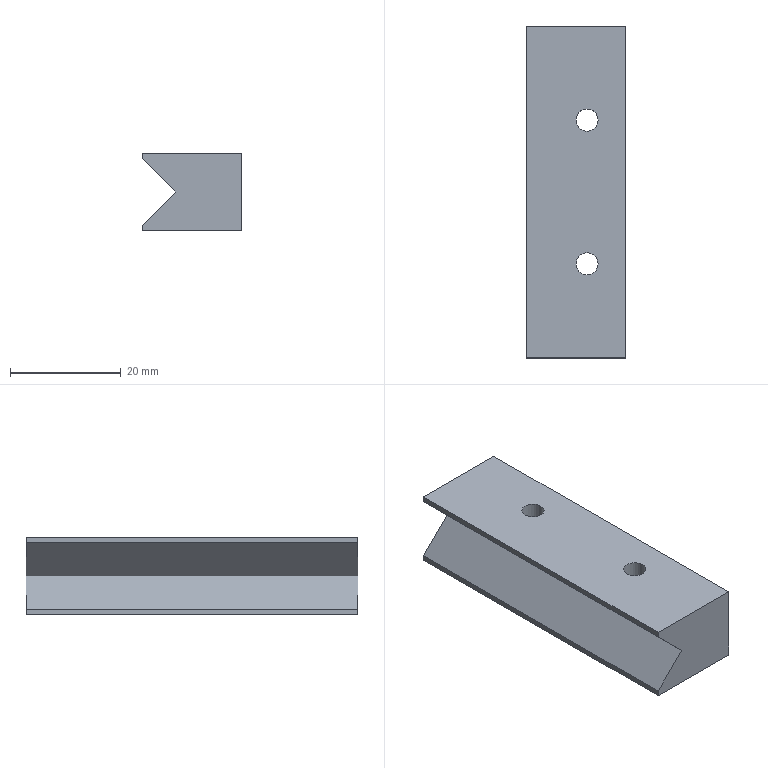Component | NX | 4_V_GUIDE | 1 solid | 15 faces | box 18 x 60 x 14 mm | volume 12264 mm3 | plane 9 | cylinder 4 | cone 2 | commonest cylinder face diameters 4 x2 4.2 x2
STEP:
#1=CARTESIAN_POINT('',(0.,0.,0.));
#2=DIRECTION('',(0.,0.,1.));
#3=DIRECTION('',(1.,0.,0.));
#4=AXIS2_PLACEMENT_3D('',#1,#2,#3);
#5=CARTESIAN_POINT('',(46.,30.,28.));
#6=VERTEX_POINT('',#5);
#7=CARTESIAN_POINT('',(46.,30.,27.));
#8=VERTEX_POINT('',#7);
#9=CARTESIAN_POINT('',(46.,30.,28.));
#10=DIRECTION('',(0.,0.,-1.));
#11=VECTOR('',#10,1.);
#12=LINE('',#9,#11);
#13=CARTESIAN_POINT('',(46.,30.,28.));
#14=DIRECTION('',(-1.,0.,0.));
#15=DIRECTION('',(0.,0.,-1.));
#16=AXIS2_PLACEMENT_3D('',#13,#14,#15);
#17=PLANE('',#16);
#18=CARTESIAN_POINT('',(0.,0.));
#19=DIRECTION('',(1.,0.));
#20=VECTOR('',#19,1.);
#21=LINE('',#18,#20);
#22=(GEOMETRIC_REPRESENTATION_CONTEXT(2)PARAMETRIC_REPRESENTATION_CONTEXT()REPRESENTATION_CONTEXT('',''));
#23=DEFINITIONAL_REPRESENTATION('',(#21),#22);
#24=PCURVE('',#17,#23);
#25=CARTESIAN_POINT('',(64.,30.,21.));
#26=DIRECTION('',(0.,-1.,0.));
#27=DIRECTION('',(-1.,0.,0.));
#28=AXIS2_PLACEMENT_3D('',#25,#26,#27);
#29=PLANE('',#28);
#30=CARTESIAN_POINT('',(18.,-7.));
#31=DIRECTION('',(0.,1.));
#32=VECTOR('',#31,1.);
#33=LINE('',#30,#32);
#34=(GEOMETRIC_REPRESENTATION_CONTEXT(2)PARAMETRIC_REPRESENTATION_CONTEXT()REPRESENTATION_CONTEXT('',''));
#35=DEFINITIONAL_REPRESENTATION('',(#33),#34);
#36=PCURVE('',#29,#35);
#37=SURFACE_CURVE('',#12,(#24,#36),.PCURVE_S1.);
#38=EDGE_CURVE('',#6,#8,#37,.T.);
#39=ORIENTED_EDGE('',*,*,#38,.T.);
#40=CARTESIAN_POINT('',(46.,-30.,27.));
#41=VERTEX_POINT('',#40);
#42=CARTESIAN_POINT('',(46.,55.,27.));
#43=DIRECTION('',(0.,-1.,0.));
#44=VECTOR('',#43,1.);
#45=LINE('',#42,#44);
#46=CARTESIAN_POINT('',(1.,-25.));
#47=DIRECTION('',(0.,1.));
#48=VECTOR('',#47,1.);
#49=LINE('',#46,#48);
#50=(GEOMETRIC_REPRESENTATION_CONTEXT(2)PARAMETRIC_REPRESENTATION_CONTEXT()REPRESENTATION_CONTEXT('',''));
#51=DEFINITIONAL_REPRESENTATION('',(#49),#50);
#52=PCURVE('',#17,#51);
#53=CARTESIAN_POINT('',(46.,55.,27.));
#54=DIRECTION('',(-0.7071,0.,-0.7071));
#55=DIRECTION('',(0.7071,0.,-0.7071));
#56=AXIS2_PLACEMENT_3D('',#53,#54,#55);
#57=PLANE('',#56);
#58=CARTESIAN_POINT('',(0.,0.));
#59=DIRECTION('',(0.,1.));
#60=VECTOR('',#59,1.);
#61=LINE('',#58,#60);
#62=(GEOMETRIC_REPRESENTATION_CONTEXT(2)PARAMETRIC_REPRESENTATION_CONTEXT()REPRESENTATION_CONTEXT('',''));
#63=DEFINITIONAL_REPRESENTATION('',(#61),#62);
#64=PCURVE('',#57,#63);
#65=SURFACE_CURVE('',#45,(#52,#64),.PCURVE_S1.);
#66=EDGE_CURVE('',#8,#41,#65,.T.);
#67=ORIENTED_EDGE('',*,*,#66,.T.);
#68=CARTESIAN_POINT('',(46.,-30.,28.));
#69=VERTEX_POINT('',#68);
#70=CARTESIAN_POINT('',(46.,-30.,28.));
#71=DIRECTION('',(0.,0.,-1.));
#72=VECTOR('',#71,1.);
#73=LINE('',#70,#72);
#74=CARTESIAN_POINT('',(0.,60.));
#75=DIRECTION('',(1.,0.));
#76=VECTOR('',#75,1.);
#77=LINE('',#74,#76);
#78=(GEOMETRIC_REPRESENTATION_CONTEXT(2)PARAMETRIC_REPRESENTATION_CONTEXT()REPRESENTATION_CONTEXT('',''));
#79=DEFINITIONAL_REPRESENTATION('',(#77),#78);
#80=PCURVE('',#17,#79);
#81=CARTESIAN_POINT('',(64.,-30.,21.));
#82=DIRECTION('',(0.,-1.,0.));
#83=DIRECTION('',(-1.,0.,0.));
#84=AXIS2_PLACEMENT_3D('',#81,#82,#83);
#85=PLANE('',#84);
#86=CARTESIAN_POINT('',(18.,-7.));
#87=DIRECTION('',(0.,1.));
#88=VECTOR('',#87,1.);
#89=LINE('',#86,#88);
#90=(GEOMETRIC_REPRESENTATION_CONTEXT(2)PARAMETRIC_REPRESENTATION_CONTEXT()REPRESENTATION_CONTEXT('',''));
#91=DEFINITIONAL_REPRESENTATION('',(#89),#90);
#92=PCURVE('',#85,#91);
#93=SURFACE_CURVE('',#73,(#80,#92),.PCURVE_S1.);
#94=EDGE_CURVE('',#69,#41,#93,.T.);
#95=ORIENTED_EDGE('',*,*,#94,.F.);
#96=CARTESIAN_POINT('',(46.,30.,28.));
#97=DIRECTION('',(0.,-1.,0.));
#98=VECTOR('',#97,1.);
#99=LINE('',#96,#98);
#100=CARTESIAN_POINT('',(0.,0.));
#101=DIRECTION('',(0.,1.));
#102=VECTOR('',#101,1.);
#103=LINE('',#100,#102);
#104=(GEOMETRIC_REPRESENTATION_CONTEXT(2)PARAMETRIC_REPRESENTATION_CONTEXT()REPRESENTATION_CONTEXT('',''));
#105=DEFINITIONAL_REPRESENTATION('',(#103),#104);
#106=PCURVE('',#17,#105);
#107=CARTESIAN_POINT('',(64.,30.,28.));
#108=DIRECTION('',(-0.,0.,1.));
#109=DIRECTION('',(-1.,0.,-0.));
#110=AXIS2_PLACEMENT_3D('',#107,#108,#109);
#111=PLANE('',#110);
#112=CARTESIAN_POINT('',(18.,0.));
#113=DIRECTION('',(0.,1.));
#114=VECTOR('',#113,1.);
#115=LINE('',#112,#114);
#116=(GEOMETRIC_REPRESENTATION_CONTEXT(2)PARAMETRIC_REPRESENTATION_CONTEXT()REPRESENTATION_CONTEXT('',''));
#117=DEFINITIONAL_REPRESENTATION('',(#115),#116);
#118=PCURVE('',#111,#117);
#119=SURFACE_CURVE('',#99,(#106,#118),.PCURVE_S1.);
#120=EDGE_CURVE('',#6,#69,#119,.T.);
#121=ORIENTED_EDGE('',*,*,#120,.F.);
#122=EDGE_LOOP('',(#39,#67,#95,#121));
#123=FACE_BOUND('',#122,.T.);
#124=ADVANCED_FACE('',(#123),#17,.T.);
#125=CARTESIAN_POINT('',(52.,30.,21.));
#126=VERTEX_POINT('',#125);
#127=CARTESIAN_POINT('',(58.,30.,15.));
#128=DIRECTION('',(0.7071,0.,-0.7071));
#129=VECTOR('',#128,1.);
#130=LINE('',#127,#129);
#131=CARTESIAN_POINT('',(6.,6.));
#132=DIRECTION('',(-0.7071,0.7071));
#133=VECTOR('',#132,1.);
#134=LINE('',#131,#133);
#135=(GEOMETRIC_REPRESENTATION_CONTEXT(2)PARAMETRIC_REPRESENTATION_CONTEXT()REPRESENTATION_CONTEXT('',''));
#136=DEFINITIONAL_REPRESENTATION('',(#134),#135);
#137=PCURVE('',#29,#136);
#138=CARTESIAN_POINT('',(16.971,25.));
#139=DIRECTION('',(1.,0.));
#140=VECTOR('',#139,1.);
#141=LINE('',#138,#140);
#142=(GEOMETRIC_REPRESENTATION_CONTEXT(2)PARAMETRIC_REPRESENTATION_CONTEXT()REPRESENTATION_CONTEXT('',''));
#143=DEFINITIONAL_REPRESENTATION('',(#141),#142);
#144=PCURVE('',#57,#143);
#145=SURFACE_CURVE('',#130,(#137,#144),.PCURVE_S1.);
#146=EDGE_CURVE('',#8,#126,#145,.T.);
#147=ORIENTED_EDGE('',*,*,#146,.F.);
#148=ORIENTED_EDGE('',*,*,#38,.F.);
#149=CARTESIAN_POINT('',(64.,30.,28.));
#150=VERTEX_POINT('',#149);
#151=CARTESIAN_POINT('',(64.,30.,28.));
#152=DIRECTION('',(-1.,0.,-0.));
#153=VECTOR('',#152,1.);
#154=LINE('',#151,#153);
#155=CARTESIAN_POINT('',(0.,-7.));
#156=DIRECTION('',(1.,0.));
#157=VECTOR('',#156,1.);
#158=LINE('',#155,#157);
#159=(GEOMETRIC_REPRESENTATION_CONTEXT(2)PARAMETRIC_REPRESENTATION_CONTEXT()REPRESENTATION_CONTEXT('',''));
#160=DEFINITIONAL_REPRESENTATION('',(#158),#159);
#161=PCURVE('',#29,#160);
#162=CARTESIAN_POINT('',(0.,0.));
#163=DIRECTION('',(1.,0.));
#164=VECTOR('',#163,1.);
#165=LINE('',#162,#164);
#166=(GEOMETRIC_REPRESENTATION_CONTEXT(2)PARAMETRIC_REPRESENTATION_CONTEXT()REPRESENTATION_CONTEXT('',''));
#167=DEFINITIONAL_REPRESENTATION('',(#165),#166);
#168=PCURVE('',#111,#167);
#169=SURFACE_CURVE('',#154,(#161,#168),.PCURVE_S1.);
#170=EDGE_CURVE('',#150,#6,#169,.T.);
#171=ORIENTED_EDGE('',*,*,#170,.F.);
#172=CARTESIAN_POINT('',(64.,30.,14.));
#173=VERTEX_POINT('',#172);
#174=CARTESIAN_POINT('',(64.,30.,14.));
#175=DIRECTION('',(0.,0.,1.));
#176=VECTOR('',#175,1.);
#177=LINE('',#174,#176);
#178=CARTESIAN_POINT('',(0.,7.));
#179=DIRECTION('',(-0.,-1.));
#180=VECTOR('',#179,1.);
#181=LINE('',#178,#180);
#182=(GEOMETRIC_REPRESENTATION_CONTEXT(2)PARAMETRIC_REPRESENTATION_CONTEXT()REPRESENTATION_CONTEXT('',''));
#183=DEFINITIONAL_REPRESENTATION('',(#181),#182);
#184=PCURVE('',#29,#183);
#185=CARTESIAN_POINT('',(64.,30.,14.));
#186=DIRECTION('',(1.,0.,-0.));
#187=DIRECTION('',(0.,0.,1.));
#188=AXIS2_PLACEMENT_3D('',#185,#186,#187);
#189=PLANE('',#188);
#190=CARTESIAN_POINT('',(0.,0.));
#191=DIRECTION('',(1.,0.));
#192=VECTOR('',#191,1.);
#193=LINE('',#190,#192);
#194=(GEOMETRIC_REPRESENTATION_CONTEXT(2)PARAMETRIC_REPRESENTATION_CONTEXT()REPRESENTATION_CONTEXT('',''));
#195=DEFINITIONAL_REPRESENTATION('',(#193),#194);
#196=PCURVE('',#189,#195);
#197=SURFACE_CURVE('',#177,(#184,#196),.PCURVE_S1.);
#198=EDGE_CURVE('',#173,#150,#197,.T.);
#199=ORIENTED_EDGE('',*,*,#198,.F.);
#200=CARTESIAN_POINT('',(46.,30.,14.));
#201=VERTEX_POINT('',#200);
#202=CARTESIAN_POINT('',(46.,30.,14.));
#203=DIRECTION('',(1.,0.,-0.));
#204=VECTOR('',#203,1.);
#205=LINE('',#202,#204);
#206=CARTESIAN_POINT('',(18.,7.));
#207=DIRECTION('',(-1.,0.));
#208=VECTOR('',#207,1.);
#209=LINE('',#206,#208);
#210=(GEOMETRIC_REPRESENTATION_CONTEXT(2)PARAMETRIC_REPRESENTATION_CONTEXT()REPRESENTATION_CONTEXT('',''));
#211=DEFINITIONAL_REPRESENTATION('',(#209),#210);
#212=PCURVE('',#29,#211);
#213=CARTESIAN_POINT('',(46.,30.,14.));
#214=DIRECTION('',(-0.,0.,-1.));
#215=DIRECTION('',(1.,0.,-0.));
#216=AXIS2_PLACEMENT_3D('',#213,#214,#215);
#217=PLANE('',#216);
#218=CARTESIAN_POINT('',(0.,0.));
#219=DIRECTION('',(1.,0.));
#220=VECTOR('',#219,1.);
#221=LINE('',#218,#220);
#222=(GEOMETRIC_REPRESENTATION_CONTEXT(2)PARAMETRIC_REPRESENTATION_CONTEXT()REPRESENTATION_CONTEXT('',''));
#223=DEFINITIONAL_REPRESENTATION('',(#221),#222);
#224=PCURVE('',#217,#223);
#225=SURFACE_CURVE('',#205,(#212,#224),.PCURVE_S1.);
#226=EDGE_CURVE('',#201,#173,#225,.T.);
#227=ORIENTED_EDGE('',*,*,#226,.F.);
#228=CARTESIAN_POINT('',(46.,30.,15.));
#229=VERTEX_POINT('',#228);
#230=CARTESIAN_POINT('',(46.,30.,28.));
#231=DIRECTION('',(0.,0.,-1.));
#232=VECTOR('',#231,1.);
#233=LINE('',#230,#232);
#234=CARTESIAN_POINT('',(18.,-7.));
#235=DIRECTION('',(0.,1.));
#236=VECTOR('',#235,1.);
#237=LINE('',#234,#236);
#238=(GEOMETRIC_REPRESENTATION_CONTEXT(2)PARAMETRIC_REPRESENTATION_CONTEXT()REPRESENTATION_CONTEXT('',''));
#239=DEFINITIONAL_REPRESENTATION('',(#237),#238);
#240=PCURVE('',#29,#239);
#241=CARTESIAN_POINT('',(46.,30.,28.));
#242=DIRECTION('',(-1.,0.,0.));
#243=DIRECTION('',(0.,0.,-1.));
#244=AXIS2_PLACEMENT_3D('',#241,#242,#243);
#245=PLANE('',#244);
#246=CARTESIAN_POINT('',(0.,0.));
#247=DIRECTION('',(1.,0.));
#248=VECTOR('',#247,1.);
#249=LINE('',#246,#248);
#250=(GEOMETRIC_REPRESENTATION_CONTEXT(2)PARAMETRIC_REPRESENTATION_CONTEXT()REPRESENTATION_CONTEXT('',''));
#251=DEFINITIONAL_REPRESENTATION('',(#249),#250);
#252=PCURVE('',#245,#251);
#253=SURFACE_CURVE('',#233,(#240,#252),.PCURVE_S1.);
#254=EDGE_CURVE('',#229,#201,#253,.T.);
#255=ORIENTED_EDGE('',*,*,#254,.F.);
#256=CARTESIAN_POINT('',(58.,30.,27.));
#257=DIRECTION('',(-0.7071,0.,-0.7071));
#258=VECTOR('',#257,1.);
#259=LINE('',#256,#258);
#260=CARTESIAN_POINT('',(6.,-6.));
#261=DIRECTION('',(0.7071,0.7071));
#262=VECTOR('',#261,1.);
#263=LINE('',#260,#262);
#264=(GEOMETRIC_REPRESENTATION_CONTEXT(2)PARAMETRIC_REPRESENTATION_CONTEXT()REPRESENTATION_CONTEXT('',''));
#265=DEFINITIONAL_REPRESENTATION('',(#263),#264);
#266=PCURVE('',#29,#265);
#267=CARTESIAN_POINT('',(52.,55.,21.));
#268=DIRECTION('',(-0.7071,0.,0.7071));
#269=DIRECTION('',(-0.7071,0.,-0.7071));
#270=AXIS2_PLACEMENT_3D('',#267,#268,#269);
#271=PLANE('',#270);
#272=CARTESIAN_POINT('',(-8.485,25.));
#273=DIRECTION('',(1.,0.));
#274=VECTOR('',#273,1.);
#275=LINE('',#272,#274);
#276=(GEOMETRIC_REPRESENTATION_CONTEXT(2)PARAMETRIC_REPRESENTATION_CONTEXT()REPRESENTATION_CONTEXT('',''));
#277=DEFINITIONAL_REPRESENTATION('',(#275),#276);
#278=PCURVE('',#271,#277);
#279=SURFACE_CURVE('',#259,(#266,#278),.PCURVE_S1.);
#280=EDGE_CURVE('',#126,#229,#279,.T.);
#281=ORIENTED_EDGE('',*,*,#280,.F.);
#282=EDGE_LOOP('',(#147,#148,#171,#199,#227,#255,#281));
#283=FACE_BOUND('',#282,.T.);
#284=ADVANCED_FACE('',(#283),#29,.F.);
#285=ORIENTED_EDGE('',*,*,#94,.T.);
#286=CARTESIAN_POINT('',(52.,-30.,21.));
#287=VERTEX_POINT('',#286);
#288=CARTESIAN_POINT('',(58.,-30.,15.));
#289=DIRECTION('',(0.7071,0.,-0.7071));
#290=VECTOR('',#289,1.);
#291=LINE('',#288,#290);
#292=CARTESIAN_POINT('',(6.,6.));
#293=DIRECTION('',(-0.7071,0.7071));
#294=VECTOR('',#293,1.);
#295=LINE('',#292,#294);
#296=(GEOMETRIC_REPRESENTATION_CONTEXT(2)PARAMETRIC_REPRESENTATION_CONTEXT()REPRESENTATION_CONTEXT('',''));
#297=DEFINITIONAL_REPRESENTATION('',(#295),#296);
#298=PCURVE('',#85,#297);
#299=CARTESIAN_POINT('',(16.971,85.));
#300=DIRECTION('',(1.,0.));
#301=VECTOR('',#300,1.);
#302=LINE('',#299,#301);
#303=(GEOMETRIC_REPRESENTATION_CONTEXT(2)PARAMETRIC_REPRESENTATION_CONTEXT()REPRESENTATION_CONTEXT('',''));
#304=DEFINITIONAL_REPRESENTATION('',(#302),#303);
#305=PCURVE('',#57,#304);
#306=SURFACE_CURVE('',#291,(#298,#305),.PCURVE_S1.);
#307=EDGE_CURVE('',#41,#287,#306,.T.);
#308=ORIENTED_EDGE('',*,*,#307,.T.);
#309=CARTESIAN_POINT('',(46.,-30.,15.));
#310=VERTEX_POINT('',#309);
#311=CARTESIAN_POINT('',(58.,-30.,27.));
#312=DIRECTION('',(-0.7071,0.,-0.7071));
#313=VECTOR('',#312,1.);
#314=LINE('',#311,#313);
#315=CARTESIAN_POINT('',(6.,-6.));
#316=DIRECTION('',(0.7071,0.7071));
#317=VECTOR('',#316,1.);
#318=LINE('',#315,#317);
#319=(GEOMETRIC_REPRESENTATION_CONTEXT(2)PARAMETRIC_REPRESENTATION_CONTEXT()REPRESENTATION_CONTEXT('',''));
#320=DEFINITIONAL_REPRESENTATION('',(#318),#319);
#321=PCURVE('',#85,#320);
#322=CARTESIAN_POINT('',(-8.485,85.));
#323=DIRECTION('',(1.,0.));
#324=VECTOR('',#323,1.);
#325=LINE('',#322,#324);
#326=(GEOMETRIC_REPRESENTATION_CONTEXT(2)PARAMETRIC_REPRESENTATION_CONTEXT()REPRESENTATION_CONTEXT('',''));
#327=DEFINITIONAL_REPRESENTATION('',(#325),#326);
#328=PCURVE('',#271,#327);
#329=SURFACE_CURVE('',#314,(#321,#328),.PCURVE_S1.);
#330=EDGE_CURVE('',#287,#310,#329,.T.);
#331=ORIENTED_EDGE('',*,*,#330,.T.);
#332=CARTESIAN_POINT('',(46.,-30.,14.));
#333=VERTEX_POINT('',#332);
#334=CARTESIAN_POINT('',(46.,-30.,28.));
#335=DIRECTION('',(0.,0.,-1.));
#336=VECTOR('',#335,1.);
#337=LINE('',#334,#336);
#338=CARTESIAN_POINT('',(18.,-7.));
#339=DIRECTION('',(0.,1.));
#340=VECTOR('',#339,1.);
#341=LINE('',#338,#340);
#342=(GEOMETRIC_REPRESENTATION_CONTEXT(2)PARAMETRIC_REPRESENTATION_CONTEXT()REPRESENTATION_CONTEXT('',''));
#343=DEFINITIONAL_REPRESENTATION('',(#341),#342);
#344=PCURVE('',#85,#343);
#345=CARTESIAN_POINT('',(0.,60.));
#346=DIRECTION('',(1.,0.));
#347=VECTOR('',#346,1.);
#348=LINE('',#345,#347);
#349=(GEOMETRIC_REPRESENTATION_CONTEXT(2)PARAMETRIC_REPRESENTATION_CONTEXT()REPRESENTATION_CONTEXT('',''));
#350=DEFINITIONAL_REPRESENTATION('',(#348),#349);
#351=PCURVE('',#245,#350);
#352=SURFACE_CURVE('',#337,(#344,#351),.PCURVE_S1.);
#353=EDGE_CURVE('',#310,#333,#352,.T.);
#354=ORIENTED_EDGE('',*,*,#353,.T.);
#355=CARTESIAN_POINT('',(64.,-30.,14.));
#356=VERTEX_POINT('',#355);
#357=CARTESIAN_POINT('',(46.,-30.,14.));
#358=DIRECTION('',(1.,0.,-0.));
#359=VECTOR('',#358,1.);
#360=LINE('',#357,#359);
#361=CARTESIAN_POINT('',(18.,7.));
#362=DIRECTION('',(-1.,0.));
#363=VECTOR('',#362,1.);
#364=LINE('',#361,#363);
#365=(GEOMETRIC_REPRESENTATION_CONTEXT(2)PARAMETRIC_REPRESENTATION_CONTEXT()REPRESENTATION_CONTEXT('',''));
#366=DEFINITIONAL_REPRESENTATION('',(#364),#365);
#367=PCURVE('',#85,#366);
#368=CARTESIAN_POINT('',(0.,60.));
#369=DIRECTION('',(1.,0.));
#370=VECTOR('',#369,1.);
#371=LINE('',#368,#370);
#372=(GEOMETRIC_REPRESENTATION_CONTEXT(2)PARAMETRIC_REPRESENTATION_CONTEXT()REPRESENTATION_CONTEXT('',''));
#373=DEFINITIONAL_REPRESENTATION('',(#371),#372);
#374=PCURVE('',#217,#373);
#375=SURFACE_CURVE('',#360,(#367,#374),.PCURVE_S1.);
#376=EDGE_CURVE('',#333,#356,#375,.T.);
#377=ORIENTED_EDGE('',*,*,#376,.T.);
#378=CARTESIAN_POINT('',(64.,-30.,28.));
#379=VERTEX_POINT('',#378);
#380=CARTESIAN_POINT('',(64.,-30.,14.));
#381=DIRECTION('',(0.,0.,1.));
#382=VECTOR('',#381,1.);
#383=LINE('',#380,#382);
#384=CARTESIAN_POINT('',(0.,7.));
#385=DIRECTION('',(-0.,-1.));
#386=VECTOR('',#385,1.);
#387=LINE('',#384,#386);
#388=(GEOMETRIC_REPRESENTATION_CONTEXT(2)PARAMETRIC_REPRESENTATION_CONTEXT()REPRESENTATION_CONTEXT('',''));
#389=DEFINITIONAL_REPRESENTATION('',(#387),#388);
#390=PCURVE('',#85,#389);
#391=CARTESIAN_POINT('',(0.,60.));
#392=DIRECTION('',(1.,0.));
#393=VECTOR('',#392,1.);
#394=LINE('',#391,#393);
#395=(GEOMETRIC_REPRESENTATION_CONTEXT(2)PARAMETRIC_REPRESENTATION_CONTEXT()REPRESENTATION_CONTEXT('',''));
#396=DEFINITIONAL_REPRESENTATION('',(#394),#395);
#397=PCURVE('',#189,#396);
#398=SURFACE_CURVE('',#383,(#390,#397),.PCURVE_S1.);
#399=EDGE_CURVE('',#356,#379,#398,.T.);
#400=ORIENTED_EDGE('',*,*,#399,.T.);
#401=CARTESIAN_POINT('',(64.,-30.,28.));
#402=DIRECTION('',(-1.,0.,-0.));
#403=VECTOR('',#402,1.);
#404=LINE('',#401,#403);
#405=CARTESIAN_POINT('',(0.,-7.));
#406=DIRECTION('',(1.,0.));
#407=VECTOR('',#406,1.);
#408=LINE('',#405,#407);
#409=(GEOMETRIC_REPRESENTATION_CONTEXT(2)PARAMETRIC_REPRESENTATION_CONTEXT()REPRESENTATION_CONTEXT('',''));
#410=DEFINITIONAL_REPRESENTATION('',(#408),#409);
#411=PCURVE('',#85,#410);
#412=CARTESIAN_POINT('',(0.,60.));
#413=DIRECTION('',(1.,0.));
#414=VECTOR('',#413,1.);
#415=LINE('',#412,#414);
#416=(GEOMETRIC_REPRESENTATION_CONTEXT(2)PARAMETRIC_REPRESENTATION_CONTEXT()REPRESENTATION_CONTEXT('',''));
#417=DEFINITIONAL_REPRESENTATION('',(#415),#416);
#418=PCURVE('',#111,#417);
#419=SURFACE_CURVE('',#404,(#411,#418),.PCURVE_S1.);
#420=EDGE_CURVE('',#379,#69,#419,.T.);
#421=ORIENTED_EDGE('',*,*,#420,.T.);
#422=EDGE_LOOP('',(#285,#308,#331,#354,#377,#400,#421));
#423=FACE_BOUND('',#422,.T.);
#424=ADVANCED_FACE('',(#423),#85,.T.);
#425=CARTESIAN_POINT('',(55.,-13.,28.));
#426=VERTEX_POINT('',#425);
#427=CARTESIAN_POINT('',(57.,-13.,28.));
#428=DIRECTION('',(-0.,0.,1.));
#429=DIRECTION('',(-1.,0.,-0.));
#430=AXIS2_PLACEMENT_3D('',#427,#428,#429);
#431=CIRCLE('',#430,2.);
#432=CARTESIAN_POINT('',(7.,43.));
#433=DIRECTION('',(1.,0.));
#434=AXIS2_PLACEMENT_2D('',#432,#433);
#435=CIRCLE('',#434,2.);
#436=(GEOMETRIC_REPRESENTATION_CONTEXT(2)PARAMETRIC_REPRESENTATION_CONTEXT()REPRESENTATION_CONTEXT('',''));
#437=DEFINITIONAL_REPRESENTATION('',(#435),#436);
#438=PCURVE('',#111,#437);
#439=CARTESIAN_POINT('',(57.,-13.,14.));
#440=DIRECTION('',(0.,0.,1.));
#441=DIRECTION('',(-1.,0.,0.));
#442=AXIS2_PLACEMENT_3D('',#439,#440,#441);
#443=CYLINDRICAL_SURFACE('',#442,2.);
#444=CARTESIAN_POINT('',(0.,14.));
#445=DIRECTION('',(1.,0.));
#446=VECTOR('',#445,1.);
#447=LINE('',#444,#446);
#448=(GEOMETRIC_REPRESENTATION_CONTEXT(2)PARAMETRIC_REPRESENTATION_CONTEXT()REPRESENTATION_CONTEXT('',''));
#449=DEFINITIONAL_REPRESENTATION('',(#447),#448);
#450=PCURVE('',#443,#449);
#451=SURFACE_CURVE('',#431,(#438,#450),.PCURVE_S1.);
#452=EDGE_CURVE('',#426,#426,#451,.T.);
#453=ORIENTED_EDGE('',*,*,#452,.F.);
#454=EDGE_LOOP('',(#453));
#455=FACE_BOUND('',#454,.T.);
#456=CARTESIAN_POINT('',(55.,13.,28.));
#457=VERTEX_POINT('',#456);
#458=CARTESIAN_POINT('',(57.,13.,28.));
#459=DIRECTION('',(-0.,0.,1.));
#460=DIRECTION('',(-1.,0.,-0.));
#461=AXIS2_PLACEMENT_3D('',#458,#459,#460);
#462=CIRCLE('',#461,2.);
#463=CARTESIAN_POINT('',(7.,17.));
#464=DIRECTION('',(1.,0.));
#465=AXIS2_PLACEMENT_2D('',#463,#464);
#466=CIRCLE('',#465,2.);
#467=(GEOMETRIC_REPRESENTATION_CONTEXT(2)PARAMETRIC_REPRESENTATION_CONTEXT()REPRESENTATION_CONTEXT('',''));
#468=DEFINITIONAL_REPRESENTATION('',(#466),#467);
#469=PCURVE('',#111,#468);
#470=CARTESIAN_POINT('',(57.,13.,14.));
#471=DIRECTION('',(0.,0.,1.));
#472=DIRECTION('',(-1.,0.,0.));
#473=AXIS2_PLACEMENT_3D('',#470,#471,#472);
#474=CYLINDRICAL_SURFACE('',#473,2.);
#475=CARTESIAN_POINT('',(0.,14.));
#476=DIRECTION('',(1.,0.));
#477=VECTOR('',#476,1.);
#478=LINE('',#475,#477);
#479=(GEOMETRIC_REPRESENTATION_CONTEXT(2)PARAMETRIC_REPRESENTATION_CONTEXT()REPRESENTATION_CONTEXT('',''));
#480=DEFINITIONAL_REPRESENTATION('',(#478),#479);
#481=PCURVE('',#474,#480);
#482=SURFACE_CURVE('',#462,(#469,#481),.PCURVE_S1.);
#483=EDGE_CURVE('',#457,#457,#482,.T.);
#484=ORIENTED_EDGE('',*,*,#483,.F.);
#485=EDGE_LOOP('',(#484));
#486=FACE_BOUND('',#485,.T.);
#487=ORIENTED_EDGE('',*,*,#420,.F.);
#488=CARTESIAN_POINT('',(64.,30.,28.));
#489=DIRECTION('',(0.,-1.,0.));
#490=VECTOR('',#489,1.);
#491=LINE('',#488,#490);
#492=CARTESIAN_POINT('',(0.,0.));
#493=DIRECTION('',(0.,1.));
#494=VECTOR('',#493,1.);
#495=LINE('',#492,#494);
#496=(GEOMETRIC_REPRESENTATION_CONTEXT(2)PARAMETRIC_REPRESENTATION_CONTEXT()REPRESENTATION_CONTEXT('',''));
#497=DEFINITIONAL_REPRESENTATION('',(#495),#496);
#498=PCURVE('',#111,#497);
#499=CARTESIAN_POINT('',(14.,0.));
#500=DIRECTION('',(0.,1.));
#501=VECTOR('',#500,1.);
#502=LINE('',#499,#501);
#503=(GEOMETRIC_REPRESENTATION_CONTEXT(2)PARAMETRIC_REPRESENTATION_CONTEXT()REPRESENTATION_CONTEXT('',''));
#504=DEFINITIONAL_REPRESENTATION('',(#502),#503);
#505=PCURVE('',#189,#504);
#506=SURFACE_CURVE('',#491,(#498,#505),.PCURVE_S1.);
#507=EDGE_CURVE('',#150,#379,#506,.T.);
#508=ORIENTED_EDGE('',*,*,#507,.F.);
#509=ORIENTED_EDGE('',*,*,#170,.T.);
#510=ORIENTED_EDGE('',*,*,#120,.T.);
#511=EDGE_LOOP('',(#487,#508,#509,#510));
#512=FACE_BOUND('',#511,.T.);
#513=ADVANCED_FACE('',(#455,#486,#512),#111,.T.);
#514=CARTESIAN_POINT('',(46.,55.,15.));
#515=DIRECTION('',(0.,-1.,0.));
#516=VECTOR('',#515,1.);
#517=LINE('',#514,#516);
#518=CARTESIAN_POINT('',(13.,-25.));
#519=DIRECTION('',(0.,1.));
#520=VECTOR('',#519,1.);
#521=LINE('',#518,#520);
#522=(GEOMETRIC_REPRESENTATION_CONTEXT(2)PARAMETRIC_REPRESENTATION_CONTEXT()REPRESENTATION_CONTEXT('',''));
#523=DEFINITIONAL_REPRESENTATION('',(#521),#522);
#524=PCURVE('',#245,#523);
#525=CARTESIAN_POINT('',(8.485,0.));
#526=DIRECTION('',(0.,1.));
#527=VECTOR('',#526,1.);
#528=LINE('',#525,#527);
#529=(GEOMETRIC_REPRESENTATION_CONTEXT(2)PARAMETRIC_REPRESENTATION_CONTEXT()REPRESENTATION_CONTEXT('',''));
#530=DEFINITIONAL_REPRESENTATION('',(#528),#529);
#531=PCURVE('',#271,#530);
#532=SURFACE_CURVE('',#517,(#524,#531),.PCURVE_S1.);
#533=EDGE_CURVE('',#229,#310,#532,.T.);
#534=ORIENTED_EDGE('',*,*,#533,.F.);
#535=ORIENTED_EDGE('',*,*,#254,.T.);
#536=CARTESIAN_POINT('',(46.,30.,14.));
#537=DIRECTION('',(0.,-1.,0.));
#538=VECTOR('',#537,1.);
#539=LINE('',#536,#538);
#540=CARTESIAN_POINT('',(14.,0.));
#541=DIRECTION('',(0.,1.));
#542=VECTOR('',#541,1.);
#543=LINE('',#540,#542);
#544=(GEOMETRIC_REPRESENTATION_CONTEXT(2)PARAMETRIC_REPRESENTATION_CONTEXT()REPRESENTATION_CONTEXT('',''));
#545=DEFINITIONAL_REPRESENTATION('',(#543),#544);
#546=PCURVE('',#245,#545);
#547=CARTESIAN_POINT('',(0.,0.));
#548=DIRECTION('',(0.,1.));
#549=VECTOR('',#548,1.);
#550=LINE('',#547,#549);
#551=(GEOMETRIC_REPRESENTATION_CONTEXT(2)PARAMETRIC_REPRESENTATION_CONTEXT()REPRESENTATION_CONTEXT('',''));
#552=DEFINITIONAL_REPRESENTATION('',(#550),#551);
#553=PCURVE('',#217,#552);
#554=SURFACE_CURVE('',#539,(#546,#553),.PCURVE_S1.);
#555=EDGE_CURVE('',#201,#333,#554,.T.);
#556=ORIENTED_EDGE('',*,*,#555,.T.);
#557=ORIENTED_EDGE('',*,*,#353,.F.);
#558=EDGE_LOOP('',(#534,#535,#556,#557));
#559=FACE_BOUND('',#558,.T.);
#560=ADVANCED_FACE('',(#559),#245,.T.);
#561=CARTESIAN_POINT('',(54.9,-22.,14.));
#562=VERTEX_POINT('',#561);
#563=CARTESIAN_POINT('',(57.,-22.,14.));
#564=DIRECTION('',(0.,0.,1.));
#565=DIRECTION('',(-1.,0.,0.));
#566=AXIS2_PLACEMENT_3D('',#563,#564,#565);
#567=CIRCLE('',#566,2.1);
#568=CARTESIAN_POINT('',(8.9,52.));
#569=CARTESIAN_POINT('',(8.9,55.637));
#570=CARTESIAN_POINT('',(12.05,53.819));
#571=CARTESIAN_POINT('',(15.2,52.));
#572=CARTESIAN_POINT('',(12.05,50.181));
#573=CARTESIAN_POINT('',(8.9,48.363));
#574=CARTESIAN_POINT('',(8.9,52.));
#575=(BOUNDED_CURVE()B_SPLINE_CURVE(2,(#568,#569,#570,#571,#572,#573,#574),.UNSPECIFIED.,.T.,.F.)B_SPLINE_CURVE_WITH_KNOTS((1,2,2,2,2,1),(-2.094,0.,2.094,4.189,6.283,8.378),.UNSPECIFIED.)CURVE()GEOMETRIC_REPRESENTATION_ITEM()RATIONAL_B_SPLINE_CURVE((1.,0.5,1.,0.5,1.,0.5,1.))REPRESENTATION_ITEM(''));
#576=(GEOMETRIC_REPRESENTATION_CONTEXT(2)PARAMETRIC_REPRESENTATION_CONTEXT()REPRESENTATION_CONTEXT('',''));
#577=DEFINITIONAL_REPRESENTATION('',(#575),#576);
#578=PCURVE('',#217,#577);
#579=CARTESIAN_POINT('',(57.,-22.,14.));
#580=DIRECTION('',(0.,0.,1.));
#581=DIRECTION('',(-1.,0.,0.));
#582=AXIS2_PLACEMENT_3D('',#579,#580,#581);
#583=CYLINDRICAL_SURFACE('',#582,2.1);
#584=CARTESIAN_POINT('',(0.,-0.));
#585=DIRECTION('',(1.,0.));
#586=VECTOR('',#585,1.);
#587=LINE('',#584,#586);
#588=(GEOMETRIC_REPRESENTATION_CONTEXT(2)PARAMETRIC_REPRESENTATION_CONTEXT()REPRESENTATION_CONTEXT('',''));
#589=DEFINITIONAL_REPRESENTATION('',(#587),#588);
#590=PCURVE('',#583,#589);
#591=SURFACE_CURVE('',#567,(#578,#590),.PCURVE_S1.);
#592=EDGE_CURVE('',#562,#562,#591,.T.);
#593=ORIENTED_EDGE('',*,*,#592,.T.);
#594=EDGE_LOOP('',(#593));
#595=FACE_BOUND('',#594,.T.);
#596=CARTESIAN_POINT('',(54.9,22.,14.));
#597=VERTEX_POINT('',#596);
#598=CARTESIAN_POINT('',(57.,22.,14.));
#599=DIRECTION('',(0.,0.,1.));
#600=DIRECTION('',(-1.,0.,0.));
#601=AXIS2_PLACEMENT_3D('',#598,#599,#600);
#602=CIRCLE('',#601,2.1);
#603=CARTESIAN_POINT('',(8.9,8.));
#604=CARTESIAN_POINT('',(8.9,11.637));
#605=CARTESIAN_POINT('',(12.05,9.819));
#606=CARTESIAN_POINT('',(15.2,8.));
#607=CARTESIAN_POINT('',(12.05,6.181));
#608=CARTESIAN_POINT('',(8.9,4.363));
#609=CARTESIAN_POINT('',(8.9,8.));
#610=(BOUNDED_CURVE()B_SPLINE_CURVE(2,(#603,#604,#605,#606,#607,#608,#609),.UNSPECIFIED.,.T.,.F.)B_SPLINE_CURVE_WITH_KNOTS((1,2,2,2,2,1),(-2.094,0.,2.094,4.189,6.283,8.378),.UNSPECIFIED.)CURVE()GEOMETRIC_REPRESENTATION_ITEM()RATIONAL_B_SPLINE_CURVE((1.,0.5,1.,0.5,1.,0.5,1.))REPRESENTATION_ITEM(''));
#611=(GEOMETRIC_REPRESENTATION_CONTEXT(2)PARAMETRIC_REPRESENTATION_CONTEXT()REPRESENTATION_CONTEXT('',''));
#612=DEFINITIONAL_REPRESENTATION('',(#610),#611);
#613=PCURVE('',#217,#612);
#614=CARTESIAN_POINT('',(57.,22.,14.));
#615=DIRECTION('',(0.,0.,1.));
#616=DIRECTION('',(-1.,0.,0.));
#617=AXIS2_PLACEMENT_3D('',#614,#615,#616);
#618=CYLINDRICAL_SURFACE('',#617,2.1);
#619=CARTESIAN_POINT('',(0.,-0.));
#620=DIRECTION('',(1.,0.));
#621=VECTOR('',#620,1.);
#622=LINE('',#619,#621);
#623=(GEOMETRIC_REPRESENTATION_CONTEXT(2)PARAMETRIC_REPRESENTATION_CONTEXT()REPRESENTATION_CONTEXT('',''));
#624=DEFINITIONAL_REPRESENTATION('',(#622),#623);
#625=PCURVE('',#618,#624);
#626=SURFACE_CURVE('',#602,(#613,#625),.PCURVE_S1.);
#627=EDGE_CURVE('',#597,#597,#626,.T.);
#628=ORIENTED_EDGE('',*,*,#627,.T.);
#629=EDGE_LOOP('',(#628));
#630=FACE_BOUND('',#629,.T.);
#631=CARTESIAN_POINT('',(55.,-13.,14.));
#632=VERTEX_POINT('',#631);
#633=CARTESIAN_POINT('',(57.,-13.,14.));
#634=DIRECTION('',(0.,0.,1.));
#635=DIRECTION('',(-1.,0.,0.));
#636=AXIS2_PLACEMENT_3D('',#633,#634,#635);
#637=CIRCLE('',#636,2.);
#638=CARTESIAN_POINT('',(9.,43.));
#639=CARTESIAN_POINT('',(9.,46.464));
#640=CARTESIAN_POINT('',(12.,44.732));
#641=CARTESIAN_POINT('',(15.,43.));
#642=CARTESIAN_POINT('',(12.,41.268));
#643=CARTESIAN_POINT('',(9.,39.536));
#644=CARTESIAN_POINT('',(9.,43.));
#645=(BOUNDED_CURVE()B_SPLINE_CURVE(2,(#638,#639,#640,#641,#642,#643,#644),.UNSPECIFIED.,.T.,.F.)B_SPLINE_CURVE_WITH_KNOTS((1,2,2,2,2,1),(-2.094,0.,2.094,4.189,6.283,8.378),.UNSPECIFIED.)CURVE()GEOMETRIC_REPRESENTATION_ITEM()RATIONAL_B_SPLINE_CURVE((1.,0.5,1.,0.5,1.,0.5,1.))REPRESENTATION_ITEM(''));
#646=(GEOMETRIC_REPRESENTATION_CONTEXT(2)PARAMETRIC_REPRESENTATION_CONTEXT()REPRESENTATION_CONTEXT('',''));
#647=DEFINITIONAL_REPRESENTATION('',(#645),#646);
#648=PCURVE('',#217,#647);
#649=CARTESIAN_POINT('',(0.,-0.));
#650=DIRECTION('',(1.,0.));
#651=VECTOR('',#650,1.);
#652=LINE('',#649,#651);
#653=(GEOMETRIC_REPRESENTATION_CONTEXT(2)PARAMETRIC_REPRESENTATION_CONTEXT()REPRESENTATION_CONTEXT('',''));
#654=DEFINITIONAL_REPRESENTATION('',(#652),#653);
#655=PCURVE('',#443,#654);
#656=SURFACE_CURVE('',#637,(#648,#655),.PCURVE_S1.);
#657=EDGE_CURVE('',#632,#632,#656,.T.);
#658=ORIENTED_EDGE('',*,*,#657,.T.);
#659=EDGE_LOOP('',(#658));
#660=FACE_BOUND('',#659,.T.);
#661=CARTESIAN_POINT('',(55.,13.,14.));
#662=VERTEX_POINT('',#661);
#663=CARTESIAN_POINT('',(57.,13.,14.));
#664=DIRECTION('',(0.,0.,1.));
#665=DIRECTION('',(-1.,0.,0.));
#666=AXIS2_PLACEMENT_3D('',#663,#664,#665);
#667=CIRCLE('',#666,2.);
#668=CARTESIAN_POINT('',(9.,17.));
#669=CARTESIAN_POINT('',(9.,20.464));
#670=CARTESIAN_POINT('',(12.,18.732));
#671=CARTESIAN_POINT('',(15.,17.));
#672=CARTESIAN_POINT('',(12.,15.268));
#673=CARTESIAN_POINT('',(9.,13.536));
#674=CARTESIAN_POINT('',(9.,17.));
#675=(BOUNDED_CURVE()B_SPLINE_CURVE(2,(#668,#669,#670,#671,#672,#673,#674),.UNSPECIFIED.,.T.,.F.)B_SPLINE_CURVE_WITH_KNOTS((1,2,2,2,2,1),(-2.094,0.,2.094,4.189,6.283,8.378),.UNSPECIFIED.)CURVE()GEOMETRIC_REPRESENTATION_ITEM()RATIONAL_B_SPLINE_CURVE((1.,0.5,1.,0.5,1.,0.5,1.))REPRESENTATION_ITEM(''));
#676=(GEOMETRIC_REPRESENTATION_CONTEXT(2)PARAMETRIC_REPRESENTATION_CONTEXT()REPRESENTATION_CONTEXT('',''));
#677=DEFINITIONAL_REPRESENTATION('',(#675),#676);
#678=PCURVE('',#217,#677);
#679=CARTESIAN_POINT('',(0.,-0.));
#680=DIRECTION('',(1.,0.));
#681=VECTOR('',#680,1.);
#682=LINE('',#679,#681);
#683=(GEOMETRIC_REPRESENTATION_CONTEXT(2)PARAMETRIC_REPRESENTATION_CONTEXT()REPRESENTATION_CONTEXT('',''));
#684=DEFINITIONAL_REPRESENTATION('',(#682),#683);
#685=PCURVE('',#474,#684);
#686=SURFACE_CURVE('',#667,(#678,#685),.PCURVE_S1.);
#687=EDGE_CURVE('',#662,#662,#686,.T.);
#688=ORIENTED_EDGE('',*,*,#687,.T.);
#689=EDGE_LOOP('',(#688));
#690=FACE_BOUND('',#689,.T.);
#691=ORIENTED_EDGE('',*,*,#376,.F.);
#692=ORIENTED_EDGE('',*,*,#555,.F.);
#693=ORIENTED_EDGE('',*,*,#226,.T.);
#694=CARTESIAN_POINT('',(64.,30.,14.));
#695=DIRECTION('',(0.,-1.,0.));
#696=VECTOR('',#695,1.);
#697=LINE('',#694,#696);
#698=CARTESIAN_POINT('',(18.,0.));
#699=DIRECTION('',(0.,1.));
#700=VECTOR('',#699,1.);
#701=LINE('',#698,#700);
#702=(GEOMETRIC_REPRESENTATION_CONTEXT(2)PARAMETRIC_REPRESENTATION_CONTEXT()REPRESENTATION_CONTEXT('',''));
#703=DEFINITIONAL_REPRESENTATION('',(#701),#702);
#704=PCURVE('',#217,#703);
#705=CARTESIAN_POINT('',(0.,0.));
#706=DIRECTION('',(0.,1.));
#707=VECTOR('',#706,1.);
#708=LINE('',#705,#707);
#709=(GEOMETRIC_REPRESENTATION_CONTEXT(2)PARAMETRIC_REPRESENTATION_CONTEXT()REPRESENTATION_CONTEXT('',''));
#710=DEFINITIONAL_REPRESENTATION('',(#708),#709);
#711=PCURVE('',#189,#710);
#712=SURFACE_CURVE('',#697,(#704,#711),.PCURVE_S1.);
#713=EDGE_CURVE('',#173,#356,#712,.T.);
#714=ORIENTED_EDGE('',*,*,#713,.T.);
#715=EDGE_LOOP('',(#691,#692,#693,#714));
#716=FACE_BOUND('',#715,.T.);
#717=ADVANCED_FACE('',(#595,#630,#660,#690,#716),#217,.T.);
#718=ORIENTED_EDGE('',*,*,#399,.F.);
#719=ORIENTED_EDGE('',*,*,#713,.F.);
#720=ORIENTED_EDGE('',*,*,#198,.T.);
#721=ORIENTED_EDGE('',*,*,#507,.T.);
#722=EDGE_LOOP('',(#718,#719,#720,#721));
#723=FACE_BOUND('',#722,.T.);
#724=ADVANCED_FACE('',(#723),#189,.T.);
#725=ORIENTED_EDGE('',*,*,#146,.T.);
#726=CARTESIAN_POINT('',(52.,55.,21.));
#727=DIRECTION('',(0.,1.,0.));
#728=VECTOR('',#727,1.);
#729=LINE('',#726,#728);
#730=CARTESIAN_POINT('',(8.485,0.));
#731=DIRECTION('',(0.,-1.));
#732=VECTOR('',#731,1.);
#733=LINE('',#730,#732);
#734=(GEOMETRIC_REPRESENTATION_CONTEXT(2)PARAMETRIC_REPRESENTATION_CONTEXT()REPRESENTATION_CONTEXT('',''));
#735=DEFINITIONAL_REPRESENTATION('',(#733),#734);
#736=PCURVE('',#57,#735);
#737=CARTESIAN_POINT('',(0.,0.));
#738=DIRECTION('',(0.,-1.));
#739=VECTOR('',#738,1.);
#740=LINE('',#737,#739);
#741=(GEOMETRIC_REPRESENTATION_CONTEXT(2)PARAMETRIC_REPRESENTATION_CONTEXT()REPRESENTATION_CONTEXT('',''));
#742=DEFINITIONAL_REPRESENTATION('',(#740),#741);
#743=PCURVE('',#271,#742);
#744=SURFACE_CURVE('',#729,(#736,#743),.PCURVE_S1.);
#745=EDGE_CURVE('',#287,#126,#744,.T.);
#746=ORIENTED_EDGE('',*,*,#745,.F.);
#747=ORIENTED_EDGE('',*,*,#307,.F.);
#748=ORIENTED_EDGE('',*,*,#66,.F.);
#749=EDGE_LOOP('',(#725,#746,#747,#748));
#750=FACE_BOUND('',#749,.T.);
#751=ADVANCED_FACE('',(#750),#57,.T.);
#752=ORIENTED_EDGE('',*,*,#280,.T.);
#753=ORIENTED_EDGE('',*,*,#533,.T.);
#754=ORIENTED_EDGE('',*,*,#330,.F.);
#755=ORIENTED_EDGE('',*,*,#745,.T.);
#756=EDGE_LOOP('',(#752,#753,#754,#755));
#757=FACE_BOUND('',#756,.T.);
#758=ADVANCED_FACE('',(#757),#271,.T.);
#759=ORIENTED_EDGE('',*,*,#483,.F.);
#760=CARTESIAN_POINT('',(55.,13.,14.));
#761=CARTESIAN_POINT('',(55.,13.,28.));
#762=B_SPLINE_CURVE_WITH_KNOTS('',1,(#760,#761),.UNSPECIFIED.,.F.,.F.,(2,2),(-0.,14.),.PIECEWISE_BEZIER_KNOTS.);
#763=CARTESIAN_POINT('',(0.,0.));
#764=DIRECTION('',(0.,1.));
#765=VECTOR('',#764,1.);
#766=LINE('',#763,#765);
#767=(GEOMETRIC_REPRESENTATION_CONTEXT(2)PARAMETRIC_REPRESENTATION_CONTEXT()REPRESENTATION_CONTEXT('',''));
#768=DEFINITIONAL_REPRESENTATION('',(#766),#767);
#769=PCURVE('',#474,#768);
#770=CARTESIAN_POINT('',(6.283,0.));
#771=DIRECTION('',(0.,1.));
#772=VECTOR('',#771,1.);
#773=LINE('',#770,#772);
#774=(GEOMETRIC_REPRESENTATION_CONTEXT(2)PARAMETRIC_REPRESENTATION_CONTEXT()REPRESENTATION_CONTEXT('',''));
#775=DEFINITIONAL_REPRESENTATION('',(#773),#774);
#776=PCURVE('',#474,#775);
#777=SEAM_CURVE('',#762,(#769,#776),.PCURVE_S1.);
#778=EDGE_CURVE('',#662,#457,#777,.T.);
#779=ORIENTED_EDGE('',*,*,#778,.F.);
#780=ORIENTED_EDGE('',*,*,#687,.T.);
#781=ORIENTED_EDGE('',*,*,#778,.T.);
#782=EDGE_LOOP('',(#759,#779,#780,#781));
#783=FACE_BOUND('',#782,.F.);
#784=ADVANCED_FACE('',(#783),#474,.F.);
#785=ORIENTED_EDGE('',*,*,#452,.F.);
#786=CARTESIAN_POINT('',(55.,-13.,14.));
#787=CARTESIAN_POINT('',(55.,-13.,28.));
#788=B_SPLINE_CURVE_WITH_KNOTS('',1,(#786,#787),.UNSPECIFIED.,.F.,.F.,(2,2),(-0.,14.),.PIECEWISE_BEZIER_KNOTS.);
#789=CARTESIAN_POINT('',(0.,0.));
#790=DIRECTION('',(0.,1.));
#791=VECTOR('',#790,1.);
#792=LINE('',#789,#791);
#793=(GEOMETRIC_REPRESENTATION_CONTEXT(2)PARAMETRIC_REPRESENTATION_CONTEXT()REPRESENTATION_CONTEXT('',''));
#794=DEFINITIONAL_REPRESENTATION('',(#792),#793);
#795=PCURVE('',#443,#794);
#796=CARTESIAN_POINT('',(6.283,0.));
#797=DIRECTION('',(0.,1.));
#798=VECTOR('',#797,1.);
#799=LINE('',#796,#798);
#800=(GEOMETRIC_REPRESENTATION_CONTEXT(2)PARAMETRIC_REPRESENTATION_CONTEXT()REPRESENTATION_CONTEXT('',''));
#801=DEFINITIONAL_REPRESENTATION('',(#799),#800);
#802=PCURVE('',#443,#801);
#803=SEAM_CURVE('',#788,(#795,#802),.PCURVE_S1.);
#804=EDGE_CURVE('',#632,#426,#803,.T.);
#805=ORIENTED_EDGE('',*,*,#804,.F.);
#806=ORIENTED_EDGE('',*,*,#657,.T.);
#807=ORIENTED_EDGE('',*,*,#804,.T.);
#808=EDGE_LOOP('',(#785,#805,#806,#807));
#809=FACE_BOUND('',#808,.F.);
#810=ADVANCED_FACE('',(#809),#443,.F.);
#811=CARTESIAN_POINT('',(59.1,22.,26.));
#812=VERTEX_POINT('',#811);
#813=CARTESIAN_POINT('',(54.9,22.,26.));
#814=VERTEX_POINT('',#813);
#815=CARTESIAN_POINT('',(57.,22.,26.));
#816=DIRECTION('',(-0.,0.,-1.));
#817=DIRECTION('',(-1.,0.,0.));
#818=AXIS2_PLACEMENT_3D('',#815,#816,#817);
#819=CIRCLE('',#818,2.1);
#820=CARTESIAN_POINT('',(57.,22.,26.));
#821=DIRECTION('',(-0.,0.,-1.));
#822=DIRECTION('',(1.,0.,-0.));
#823=AXIS2_PLACEMENT_3D('',#820,#821,#822);
#824=CONICAL_SURFACE('',#823,2.1,1.03);
#825=CARTESIAN_POINT('',(-3.142,0.));
#826=DIRECTION('',(1.,0.));
#827=VECTOR('',#826,1.);
#828=LINE('',#825,#827);
#829=(GEOMETRIC_REPRESENTATION_CONTEXT(2)PARAMETRIC_REPRESENTATION_CONTEXT()REPRESENTATION_CONTEXT('',''));
#830=DEFINITIONAL_REPRESENTATION('',(#828),#829);
#831=PCURVE('',#824,#830);
#832=CARTESIAN_POINT('',(6.283,12.));
#833=DIRECTION('',(-1.,0.));
#834=VECTOR('',#833,1.);
#835=LINE('',#832,#834);
#836=(GEOMETRIC_REPRESENTATION_CONTEXT(2)PARAMETRIC_REPRESENTATION_CONTEXT()REPRESENTATION_CONTEXT('',''));
#837=DEFINITIONAL_REPRESENTATION('',(#835),#836);
#838=PCURVE('',#618,#837);
#839=SURFACE_CURVE('',#819,(#831,#838),.PCURVE_S1.);
#840=EDGE_CURVE('',#812,#814,#839,.T.);
#841=ORIENTED_EDGE('',*,*,#840,.F.);
#842=CARTESIAN_POINT('',(57.,22.,27.262));
#843=VERTEX_POINT('',#842);
#844=CARTESIAN_POINT('',(57.,22.,27.262));
#845=CARTESIAN_POINT('',(59.1,22.,26.));
#846=B_SPLINE_CURVE_WITH_KNOTS('',1,(#844,#845),.UNSPECIFIED.,.F.,.F.,(2,2),(-2.45,0.),.PIECEWISE_BEZIER_KNOTS.);
#847=CARTESIAN_POINT('',(0.,0.));
#848=DIRECTION('',(0.,1.));
#849=VECTOR('',#848,1.);
#850=LINE('',#847,#849);
#851=(GEOMETRIC_REPRESENTATION_CONTEXT(2)PARAMETRIC_REPRESENTATION_CONTEXT()REPRESENTATION_CONTEXT('',''));
#852=DEFINITIONAL_REPRESENTATION('',(#850),#851);
#853=PCURVE('',#824,#852);
#854=CARTESIAN_POINT('',(6.283,0.));
#855=DIRECTION('',(0.,1.));
#856=VECTOR('',#855,1.);
#857=LINE('',#854,#856);
#858=(GEOMETRIC_REPRESENTATION_CONTEXT(2)PARAMETRIC_REPRESENTATION_CONTEXT()REPRESENTATION_CONTEXT('',''));
#859=DEFINITIONAL_REPRESENTATION('',(#857),#858);
#860=PCURVE('',#824,#859);
#861=SEAM_CURVE('',#846,(#853,#860),.PCURVE_S1.);
#862=EDGE_CURVE('',#843,#812,#861,.T.);
#863=ORIENTED_EDGE('',*,*,#862,.F.);
#864=ORIENTED_EDGE('',*,*,#862,.T.);
#865=CARTESIAN_POINT('',(57.,22.,26.));
#866=DIRECTION('',(-0.,0.,-1.));
#867=DIRECTION('',(-1.,0.,0.));
#868=AXIS2_PLACEMENT_3D('',#865,#866,#867);
#869=CIRCLE('',#868,2.1);
#870=CARTESIAN_POINT('',(3.142,0.));
#871=DIRECTION('',(1.,0.));
#872=VECTOR('',#871,1.);
#873=LINE('',#870,#872);
#874=(GEOMETRIC_REPRESENTATION_CONTEXT(2)PARAMETRIC_REPRESENTATION_CONTEXT()REPRESENTATION_CONTEXT('',''));
#875=DEFINITIONAL_REPRESENTATION('',(#873),#874);
#876=PCURVE('',#824,#875);
#877=CARTESIAN_POINT('',(6.283,12.));
#878=DIRECTION('',(-1.,0.));
#879=VECTOR('',#878,1.);
#880=LINE('',#877,#879);
#881=(GEOMETRIC_REPRESENTATION_CONTEXT(2)PARAMETRIC_REPRESENTATION_CONTEXT()REPRESENTATION_CONTEXT('',''));
#882=DEFINITIONAL_REPRESENTATION('',(#880),#881);
#883=PCURVE('',#618,#882);
#884=SURFACE_CURVE('',#869,(#876,#883),.PCURVE_S1.);
#885=EDGE_CURVE('',#814,#812,#884,.T.);
#886=ORIENTED_EDGE('',*,*,#885,.F.);
#887=EDGE_LOOP('',(#841,#863,#864,#886));
#888=FACE_BOUND('',#887,.F.);
#889=ADVANCED_FACE('',(#888),#824,.F.);
#890=ORIENTED_EDGE('',*,*,#840,.T.);
#891=CARTESIAN_POINT('',(54.9,22.,14.));
#892=CARTESIAN_POINT('',(54.9,22.,26.));
#893=B_SPLINE_CURVE_WITH_KNOTS('',1,(#891,#892),.UNSPECIFIED.,.F.,.F.,(2,2),(-0.,12.),.PIECEWISE_BEZIER_KNOTS.);
#894=CARTESIAN_POINT('',(0.,0.));
#895=DIRECTION('',(0.,1.));
#896=VECTOR('',#895,1.);
#897=LINE('',#894,#896);
#898=(GEOMETRIC_REPRESENTATION_CONTEXT(2)PARAMETRIC_REPRESENTATION_CONTEXT()REPRESENTATION_CONTEXT('',''));
#899=DEFINITIONAL_REPRESENTATION('',(#897),#898);
#900=PCURVE('',#618,#899);
#901=CARTESIAN_POINT('',(6.283,0.));
#902=DIRECTION('',(0.,1.));
#903=VECTOR('',#902,1.);
#904=LINE('',#901,#903);
#905=(GEOMETRIC_REPRESENTATION_CONTEXT(2)PARAMETRIC_REPRESENTATION_CONTEXT()REPRESENTATION_CONTEXT('',''));
#906=DEFINITIONAL_REPRESENTATION('',(#904),#905);
#907=PCURVE('',#618,#906);
#908=SEAM_CURVE('',#893,(#900,#907),.PCURVE_S1.);
#909=EDGE_CURVE('',#597,#814,#908,.T.);
#910=ORIENTED_EDGE('',*,*,#909,.F.);
#911=ORIENTED_EDGE('',*,*,#627,.T.);
#912=ORIENTED_EDGE('',*,*,#909,.T.);
#913=ORIENTED_EDGE('',*,*,#885,.T.);
#914=EDGE_LOOP('',(#890,#910,#911,#912,#913));
#915=FACE_BOUND('',#914,.F.);
#916=ADVANCED_FACE('',(#915),#618,.F.);
#917=CARTESIAN_POINT('',(59.1,-22.,26.));
#918=VERTEX_POINT('',#917);
#919=CARTESIAN_POINT('',(54.9,-22.,26.));
#920=VERTEX_POINT('',#919);
#921=CARTESIAN_POINT('',(57.,-22.,26.));
#922=DIRECTION('',(-0.,0.,-1.));
#923=DIRECTION('',(-1.,0.,0.));
#924=AXIS2_PLACEMENT_3D('',#921,#922,#923);
#925=CIRCLE('',#924,2.1);
#926=CARTESIAN_POINT('',(57.,-22.,26.));
#927=DIRECTION('',(-0.,0.,-1.));
#928=DIRECTION('',(1.,0.,-0.));
#929=AXIS2_PLACEMENT_3D('',#926,#927,#928);
#930=CONICAL_SURFACE('',#929,2.1,1.03);
#931=CARTESIAN_POINT('',(-3.142,0.));
#932=DIRECTION('',(1.,0.));
#933=VECTOR('',#932,1.);
#934=LINE('',#931,#933);
#935=(GEOMETRIC_REPRESENTATION_CONTEXT(2)PARAMETRIC_REPRESENTATION_CONTEXT()REPRESENTATION_CONTEXT('',''));
#936=DEFINITIONAL_REPRESENTATION('',(#934),#935);
#937=PCURVE('',#930,#936);
#938=CARTESIAN_POINT('',(6.283,12.));
#939=DIRECTION('',(-1.,0.));
#940=VECTOR('',#939,1.);
#941=LINE('',#938,#940);
#942=(GEOMETRIC_REPRESENTATION_CONTEXT(2)PARAMETRIC_REPRESENTATION_CONTEXT()REPRESENTATION_CONTEXT('',''));
#943=DEFINITIONAL_REPRESENTATION('',(#941),#942);
#944=PCURVE('',#583,#943);
#945=SURFACE_CURVE('',#925,(#937,#944),.PCURVE_S1.);
#946=EDGE_CURVE('',#918,#920,#945,.T.);
#947=ORIENTED_EDGE('',*,*,#946,.F.);
#948=CARTESIAN_POINT('',(57.,-22.,27.262));
#949=VERTEX_POINT('',#948);
#950=CARTESIAN_POINT('',(57.,-22.,27.262));
#951=CARTESIAN_POINT('',(59.1,-22.,26.));
#952=B_SPLINE_CURVE_WITH_KNOTS('',1,(#950,#951),.UNSPECIFIED.,.F.,.F.,(2,2),(-2.45,0.),.PIECEWISE_BEZIER_KNOTS.);
#953=CARTESIAN_POINT('',(0.,0.));
#954=DIRECTION('',(0.,1.));
#955=VECTOR('',#954,1.);
#956=LINE('',#953,#955);
#957=(GEOMETRIC_REPRESENTATION_CONTEXT(2)PARAMETRIC_REPRESENTATION_CONTEXT()REPRESENTATION_CONTEXT('',''));
#958=DEFINITIONAL_REPRESENTATION('',(#956),#957);
#959=PCURVE('',#930,#958);
#960=CARTESIAN_POINT('',(6.283,0.));
#961=DIRECTION('',(0.,1.));
#962=VECTOR('',#961,1.);
#963=LINE('',#960,#962);
#964=(GEOMETRIC_REPRESENTATION_CONTEXT(2)PARAMETRIC_REPRESENTATION_CONTEXT()REPRESENTATION_CONTEXT('',''));
#965=DEFINITIONAL_REPRESENTATION('',(#963),#964);
#966=PCURVE('',#930,#965);
#967=SEAM_CURVE('',#952,(#959,#966),.PCURVE_S1.);
#968=EDGE_CURVE('',#949,#918,#967,.T.);
#969=ORIENTED_EDGE('',*,*,#968,.F.);
#970=ORIENTED_EDGE('',*,*,#968,.T.);
#971=CARTESIAN_POINT('',(57.,-22.,26.));
#972=DIRECTION('',(-0.,0.,-1.));
#973=DIRECTION('',(-1.,0.,0.));
#974=AXIS2_PLACEMENT_3D('',#971,#972,#973);
#975=CIRCLE('',#974,2.1);
#976=CARTESIAN_POINT('',(3.142,0.));
#977=DIRECTION('',(1.,0.));
#978=VECTOR('',#977,1.);
#979=LINE('',#976,#978);
#980=(GEOMETRIC_REPRESENTATION_CONTEXT(2)PARAMETRIC_REPRESENTATION_CONTEXT()REPRESENTATION_CONTEXT('',''));
#981=DEFINITIONAL_REPRESENTATION('',(#979),#980);
#982=PCURVE('',#930,#981);
#983=CARTESIAN_POINT('',(6.283,12.));
#984=DIRECTION('',(-1.,0.));
#985=VECTOR('',#984,1.);
#986=LINE('',#983,#985);
#987=(GEOMETRIC_REPRESENTATION_CONTEXT(2)PARAMETRIC_REPRESENTATION_CONTEXT()REPRESENTATION_CONTEXT('',''));
#988=DEFINITIONAL_REPRESENTATION('',(#986),#987);
#989=PCURVE('',#583,#988);
#990=SURFACE_CURVE('',#975,(#982,#989),.PCURVE_S1.);
#991=EDGE_CURVE('',#920,#918,#990,.T.);
#992=ORIENTED_EDGE('',*,*,#991,.F.);
#993=EDGE_LOOP('',(#947,#969,#970,#992));
#994=FACE_BOUND('',#993,.F.);
#995=ADVANCED_FACE('',(#994),#930,.F.);
#996=ORIENTED_EDGE('',*,*,#946,.T.);
#997=CARTESIAN_POINT('',(54.9,-22.,14.));
#998=CARTESIAN_POINT('',(54.9,-22.,26.));
#999=B_SPLINE_CURVE_WITH_KNOTS('',1,(#997,#998),.UNSPECIFIED.,.F.,.F.,(2,2),(-0.,12.),.PIECEWISE_BEZIER_KNOTS.);
#1000=CARTESIAN_POINT('',(0.,0.));
#1001=DIRECTION('',(0.,1.));
#1002=VECTOR('',#1001,1.);
#1003=LINE('',#1000,#1002);
#1004=(GEOMETRIC_REPRESENTATION_CONTEXT(2)PARAMETRIC_REPRESENTATION_CONTEXT()REPRESENTATION_CONTEXT('',''));
#1005=DEFINITIONAL_REPRESENTATION('',(#1003),#1004);
#1006=PCURVE('',#583,#1005);
#1007=CARTESIAN_POINT('',(6.283,0.));
#1008=DIRECTION('',(0.,1.));
#1009=VECTOR('',#1008,1.);
#1010=LINE('',#1007,#1009);
#1011=(GEOMETRIC_REPRESENTATION_CONTEXT(2)PARAMETRIC_REPRESENTATION_CONTEXT()REPRESENTATION_CONTEXT('',''));
#1012=DEFINITIONAL_REPRESENTATION('',(#1010),#1011);
#1013=PCURVE('',#583,#1012);
#1014=SEAM_CURVE('',#999,(#1006,#1013),.PCURVE_S1.);
#1015=EDGE_CURVE('',#562,#920,#1014,.T.);
#1016=ORIENTED_EDGE('',*,*,#1015,.F.);
#1017=ORIENTED_EDGE('',*,*,#592,.T.);
#1018=ORIENTED_EDGE('',*,*,#1015,.T.);
#1019=ORIENTED_EDGE('',*,*,#991,.T.);
#1020=EDGE_LOOP('',(#996,#1016,#1017,#1018,#1019));
#1021=FACE_BOUND('',#1020,.F.);
#1022=ADVANCED_FACE('',(#1021),#583,.F.);
#1023=CLOSED_SHELL('',(#124,#284,#424,#513,#560,#717,#724,#751,#758,#784,#810,#889,#916,#995,#1022));
#1024=MANIFOLD_SOLID_BREP('',#1023);
#1025=(LENGTH_UNIT()NAMED_UNIT(*)SI_UNIT(.MILLI.,.METRE.));
#1026=UNCERTAINTY_MEASURE_WITH_UNIT(LENGTH_MEASURE(0.000005),#1025,'','');
#1027=(NAMED_UNIT(*)PLANE_ANGLE_UNIT()SI_UNIT($,.RADIAN.));
#1028=(NAMED_UNIT(*)SI_UNIT($,.STERADIAN.)SOLID_ANGLE_UNIT());
#1029=(GEOMETRIC_REPRESENTATION_CONTEXT(3)GLOBAL_UNCERTAINTY_ASSIGNED_CONTEXT((#1026))GLOBAL_UNIT_ASSIGNED_CONTEXT((#1025,#1027,#1028))REPRESENTATION_CONTEXT('',''));
#1030=ADVANCED_BREP_SHAPE_REPRESENTATION('',(#4,#1024),#1029);